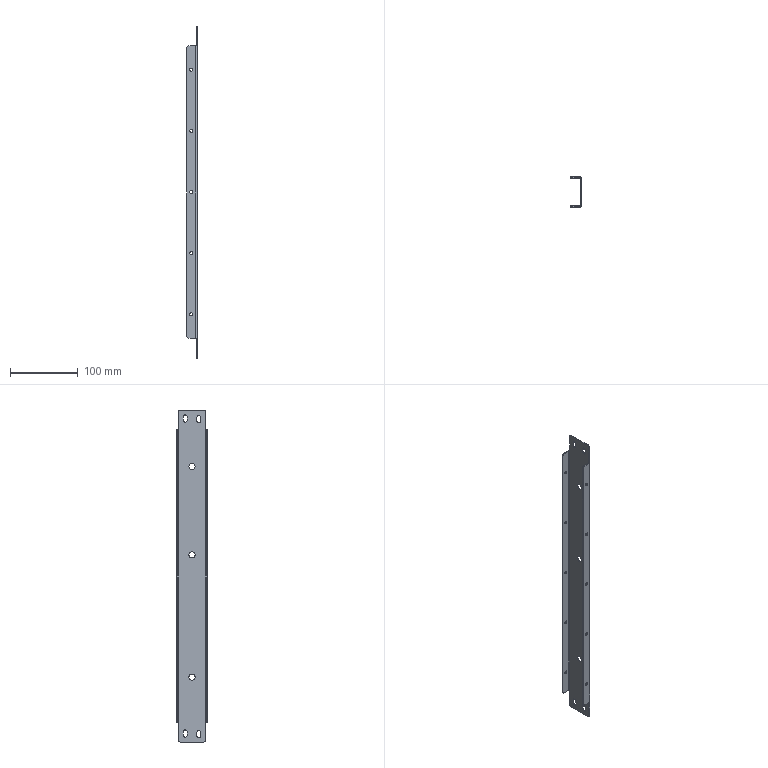Component | SolidWorks | GroundWireFixingBeam100-20 | 1 solid | 80 faces | volume 47954 mm3 | cylinder 50 | plane 30 | commonest cylinder face diameters 4.5 x20 5.5 x12 6 x8 9 x6 4.473 x2 1.473 x2